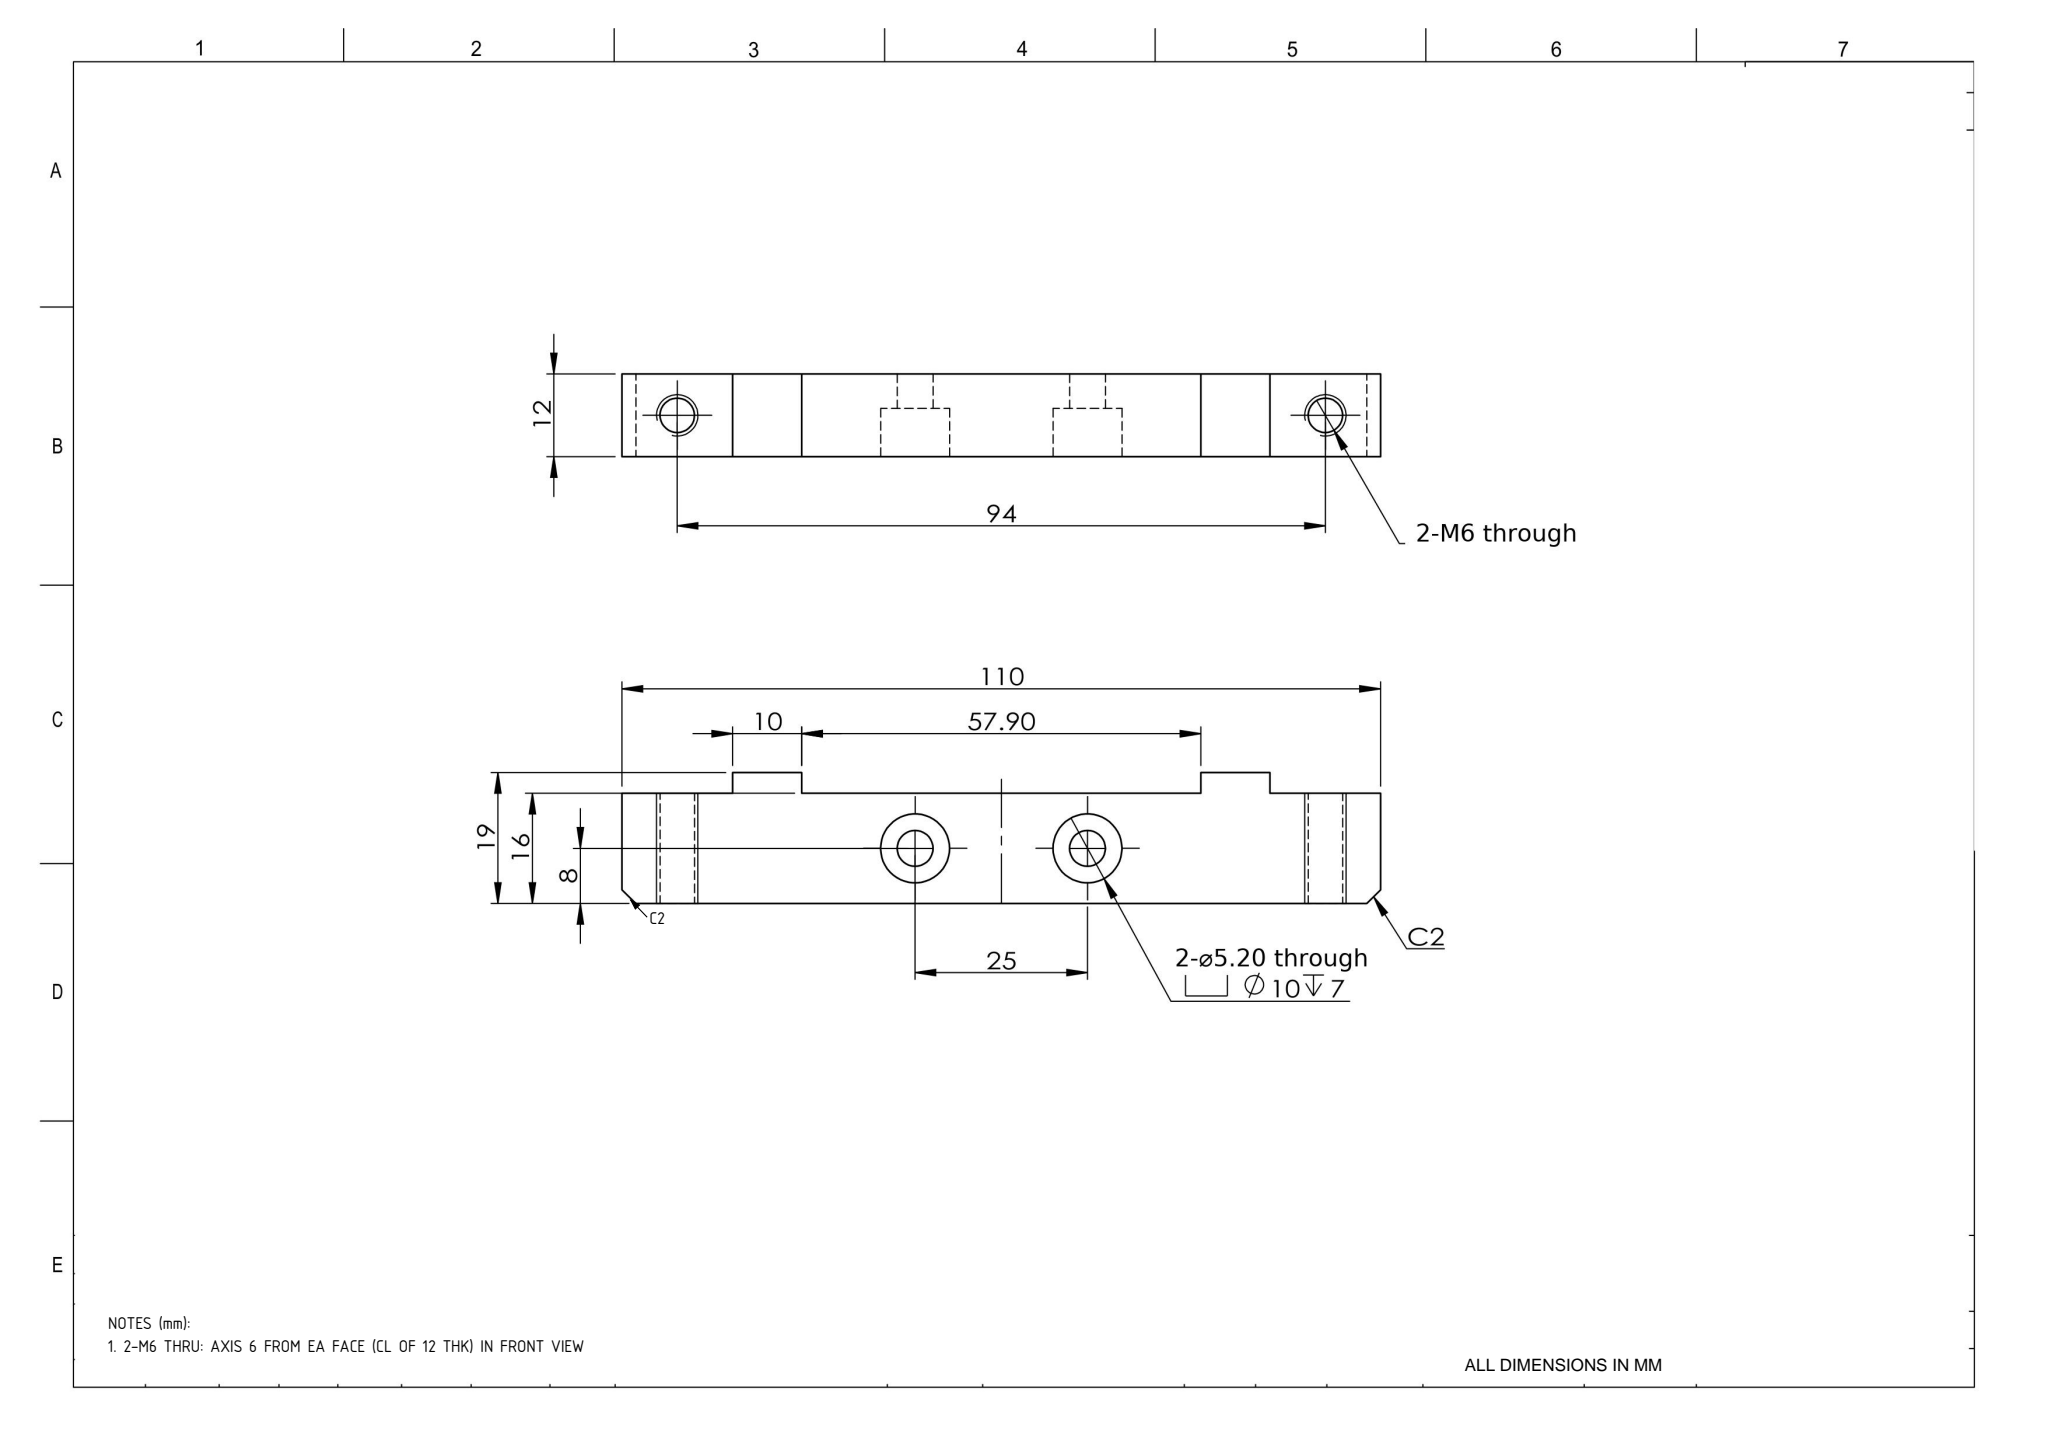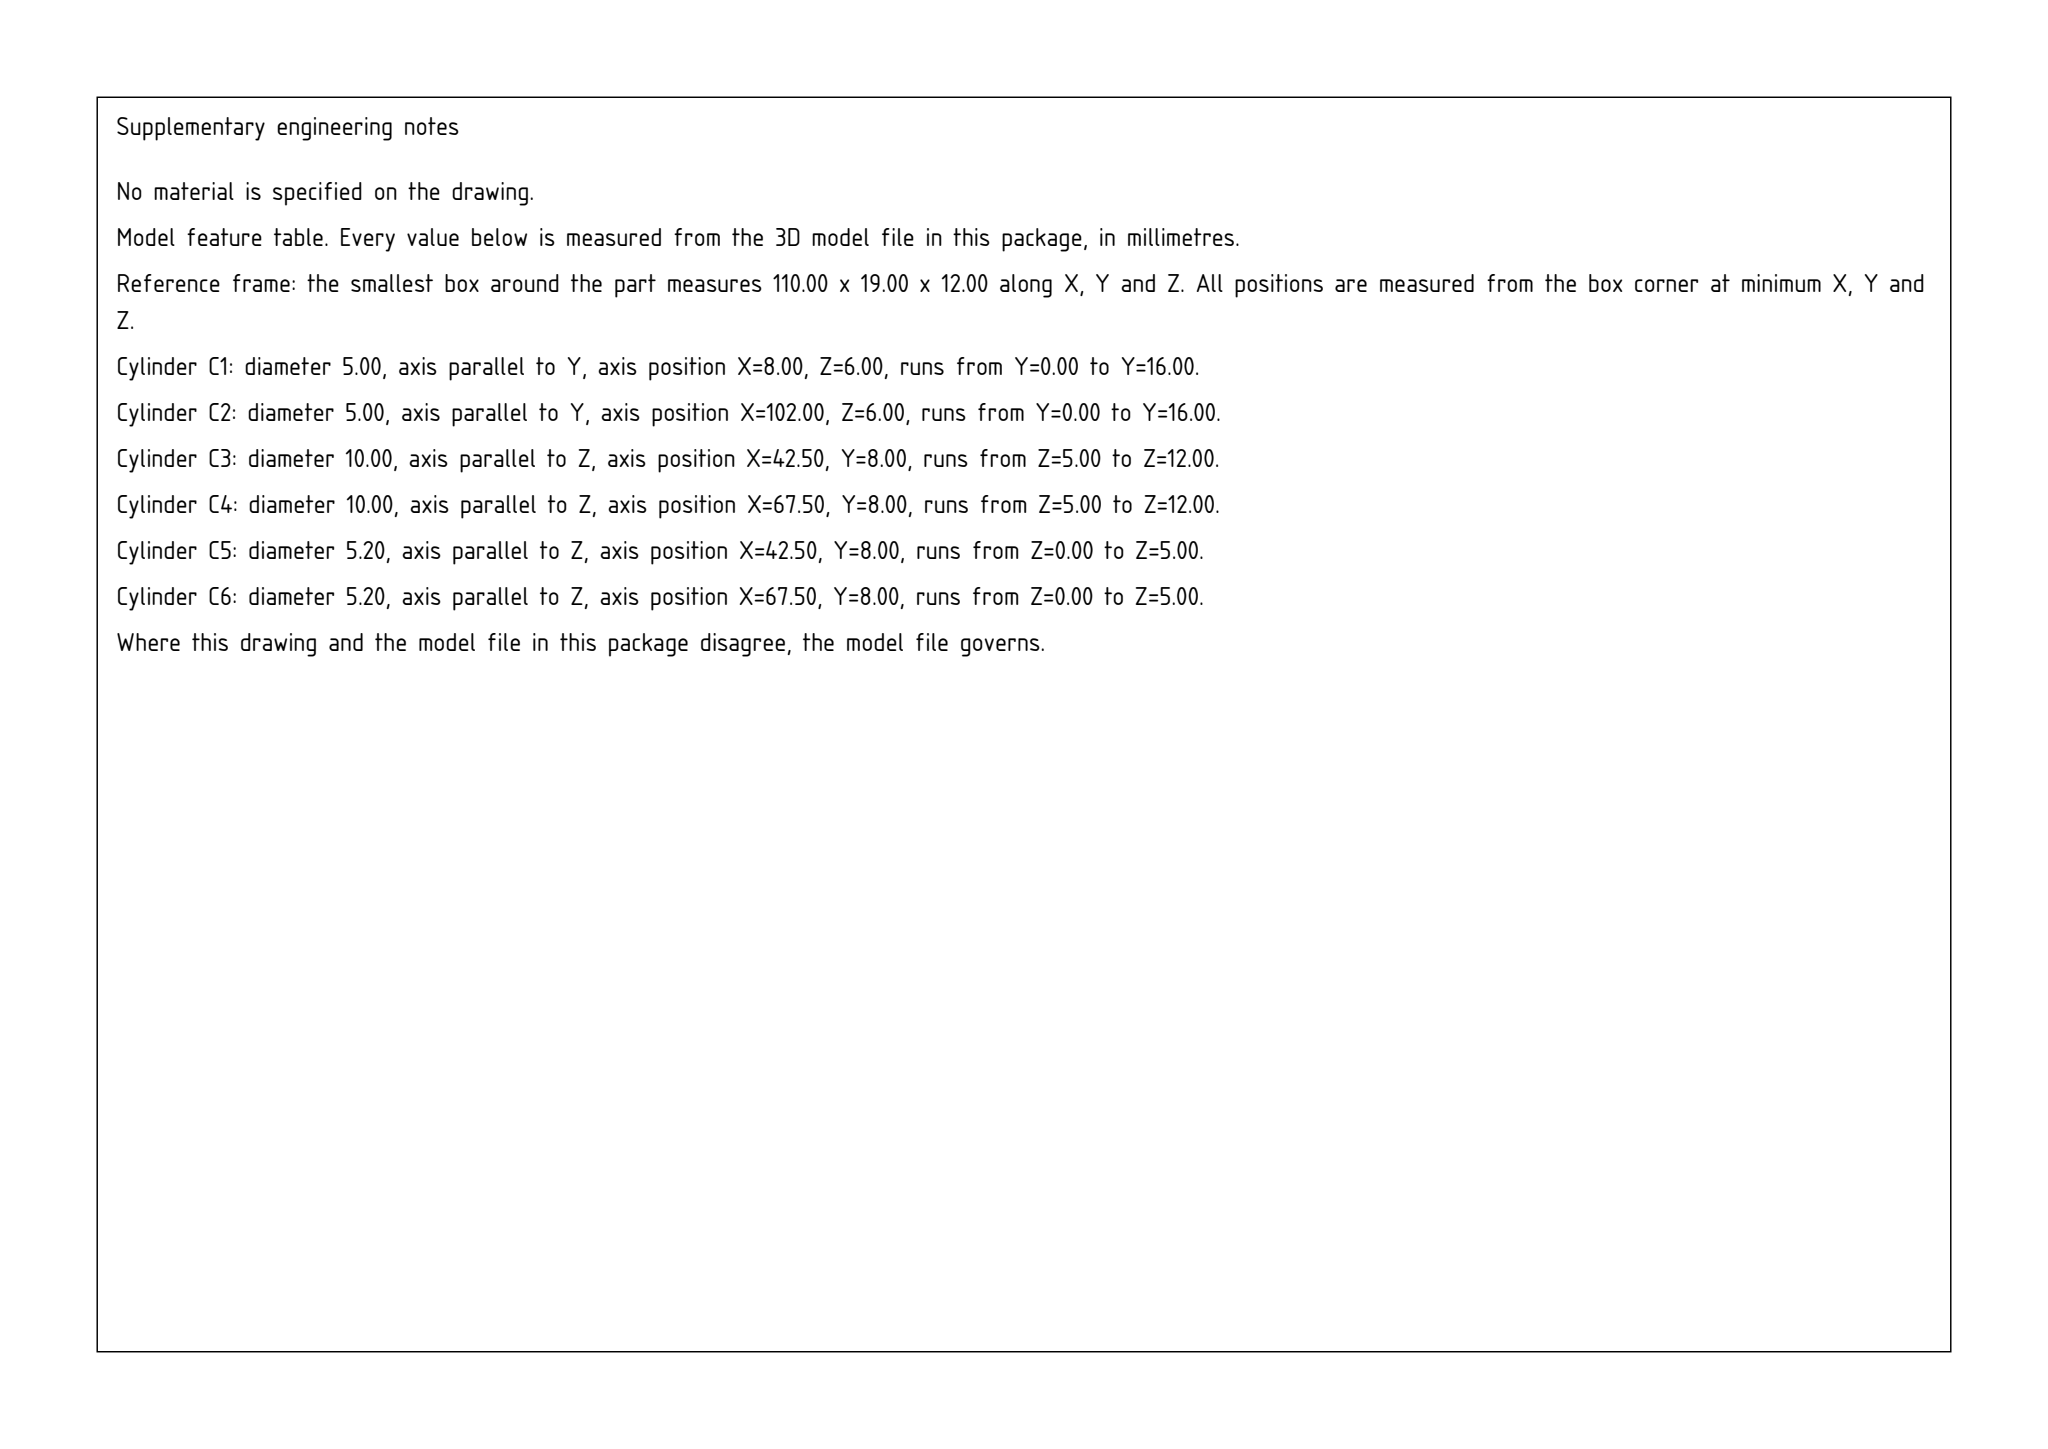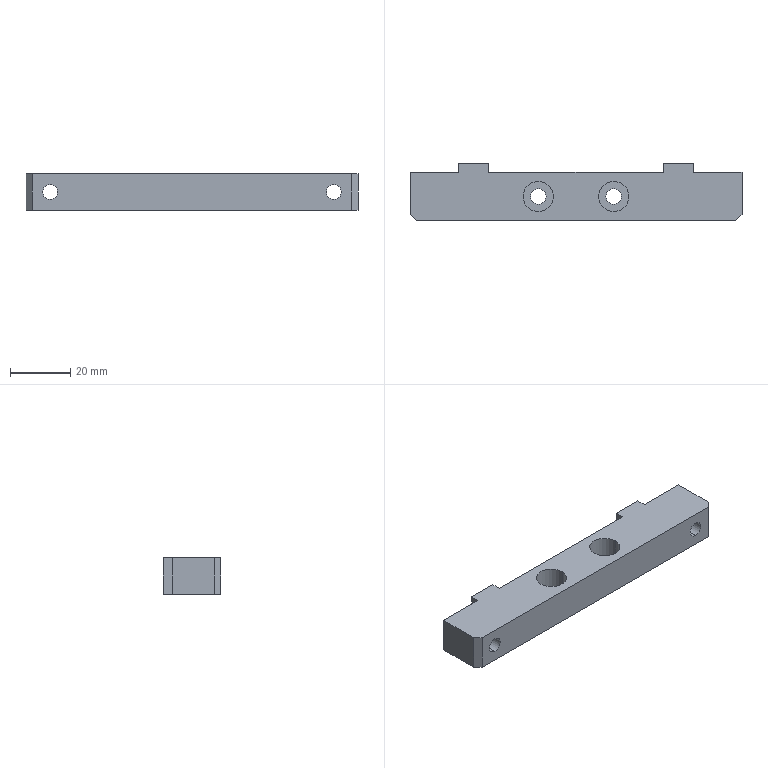Part | SolidWorks | mm | 1 solid | 30 faces | box 110 x 19 x 12 mm | volume 19852 mm3 | plane 18 | cylinder 12 | commonest cylinder face diameters 5.2 x4 5 x4 10 x4
Drawing notes:
LEFT END BOTTOM CHAMFER C2 (2 PLCS, SYM BOTH ENDS) | from the solid: Part symmetric about x=55 (bbox 110 long; steps at x=16.05/26.05 and 83.95/93.95, holes at 8/102 and 42.5/67.5); left end chamfer equals dimensioned right-end C2
2-M6 THRU: AXIS 6 FROM EA FACE (CL OF 12 THK) IN FRONT VIEW | from the solid: Ø5 y-axis holes at z=6.0; part thickness z 0-12, so axes centered